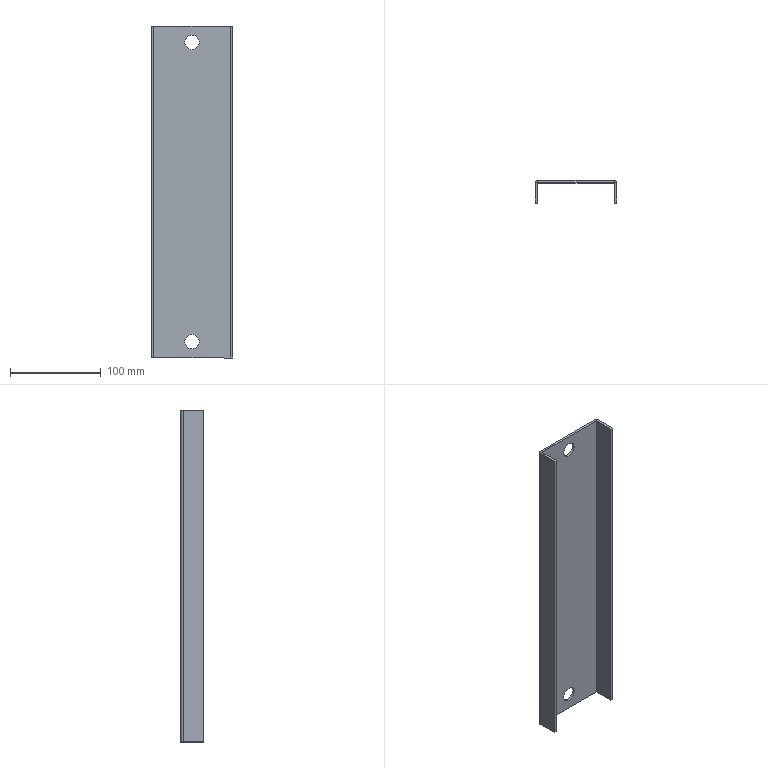Component | SolidWorks | KSHE-016.014-1 | 1 solid | 26 faces | box 90 x 25 x 366 mm | volume 121459 mm3 | plane 18 | cylinder 8 | commonest cylinder face diameters 16 x4 5.2 x2 0.2 x2
STEP:
#1=COLOUR_RGB('',0.7922,0.8196,0.9333);
#2=FILL_AREA_STYLE_COLOUR('',#1);
#3=FILL_AREA_STYLE('',(#2));
#4=SURFACE_STYLE_FILL_AREA(#3);
#5=SURFACE_SIDE_STYLE('',(#4));
#6=SURFACE_STYLE_USAGE(.BOTH.,#5);
#7=PRESENTATION_STYLE_ASSIGNMENT((#6));
#8=CARTESIAN_POINT('',(12.115,67.965,-1.713));
#9=VERTEX_POINT('',#8);
#10=CARTESIAN_POINT('',(12.115,67.965,-2.343));
#11=VERTEX_POINT('',#10);
#12=CARTESIAN_POINT('',(12.115,67.965,-2.028));
#13=DIRECTION('',(0.,1.,-0.));
#14=DIRECTION('',(0.,0.,-1.));
#15=AXIS2_PLACEMENT_3D('',#12,#13,#14);
#16=CIRCLE('',#15,0.315);
#17=EDGE_CURVE('',#9,#11,#16,.T.);
#18=ORIENTED_EDGE('',*,*,#17,.F.);
#19=CARTESIAN_POINT('',(12.115,68.064,-1.713));
#20=VERTEX_POINT('',#19);
#21=CARTESIAN_POINT('',(12.115,67.67,-1.713));
#22=DIRECTION('',(0.,1.,-0.));
#23=VECTOR('',#22,39.37);
#24=LINE('',#21,#23);
#25=EDGE_CURVE('',#9,#20,#24,.T.);
#26=ORIENTED_EDGE('',*,*,#25,.T.);
#27=CARTESIAN_POINT('',(12.115,68.064,-2.343));
#28=VERTEX_POINT('',#27);
#29=CARTESIAN_POINT('',(12.115,68.064,-2.028));
#30=DIRECTION('',(0.,1.,-0.));
#31=DIRECTION('',(0.,0.,-1.));
#32=AXIS2_PLACEMENT_3D('',#29,#30,#31);
#33=CIRCLE('',#32,0.315);
#34=EDGE_CURVE('',#20,#28,#33,.T.);
#35=ORIENTED_EDGE('',*,*,#34,.T.);
#36=CARTESIAN_POINT('',(12.115,67.67,-2.343));
#37=DIRECTION('',(0.,1.,-0.));
#38=VECTOR('',#37,39.37);
#39=LINE('',#36,#38);
#40=EDGE_CURVE('',#11,#28,#39,.T.);
#41=ORIENTED_EDGE('',*,*,#40,.F.);
#42=EDGE_LOOP('',(#18,#26,#35,#41));
#43=FACE_OUTER_BOUND('',#42,.T.);
#44=CARTESIAN_POINT('',(12.115,67.67,-2.028));
#45=DIRECTION('',(0.,1.,-0.));
#46=DIRECTION('',(0.,0.,-1.));
#47=AXIS2_PLACEMENT_3D('',#44,#45,#46);
#48=CYLINDRICAL_SURFACE('',#47,0.315);
#49=ADVANCED_FACE('',(#43),#48,.F.);
#50=CARTESIAN_POINT('',(12.115,67.965,-14.705));
#51=VERTEX_POINT('',#50);
#52=CARTESIAN_POINT('',(12.115,67.965,-15.335));
#53=VERTEX_POINT('',#52);
#54=CARTESIAN_POINT('',(12.115,67.965,-15.02));
#55=DIRECTION('',(0.,1.,-0.));
#56=DIRECTION('',(0.,0.,-1.));
#57=AXIS2_PLACEMENT_3D('',#54,#55,#56);
#58=CIRCLE('',#57,0.315);
#59=EDGE_CURVE('',#51,#53,#58,.T.);
#60=ORIENTED_EDGE('',*,*,#59,.F.);
#61=CARTESIAN_POINT('',(12.115,68.064,-14.705));
#62=VERTEX_POINT('',#61);
#63=CARTESIAN_POINT('',(12.115,67.67,-14.705));
#64=DIRECTION('',(0.,1.,-0.));
#65=VECTOR('',#64,39.37);
#66=LINE('',#63,#65);
#67=EDGE_CURVE('',#51,#62,#66,.T.);
#68=ORIENTED_EDGE('',*,*,#67,.T.);
#69=CARTESIAN_POINT('',(12.115,68.064,-15.335));
#70=VERTEX_POINT('',#69);
#71=CARTESIAN_POINT('',(12.115,68.064,-15.02));
#72=DIRECTION('',(0.,1.,-0.));
#73=DIRECTION('',(0.,0.,-1.));
#74=AXIS2_PLACEMENT_3D('',#71,#72,#73);
#75=CIRCLE('',#74,0.315);
#76=EDGE_CURVE('',#62,#70,#75,.T.);
#77=ORIENTED_EDGE('',*,*,#76,.T.);
#78=CARTESIAN_POINT('',(12.115,67.67,-15.335));
#79=DIRECTION('',(0.,1.,-0.));
#80=VECTOR('',#79,39.37);
#81=LINE('',#78,#80);
#82=EDGE_CURVE('',#53,#70,#81,.T.);
#83=ORIENTED_EDGE('',*,*,#82,.F.);
#84=EDGE_LOOP('',(#60,#68,#77,#83));
#85=FACE_OUTER_BOUND('',#84,.T.);
#86=CARTESIAN_POINT('',(12.115,67.67,-15.02));
#87=DIRECTION('',(0.,1.,-0.));
#88=DIRECTION('',(0.,0.,-1.));
#89=AXIS2_PLACEMENT_3D('',#86,#87,#88);
#90=CYLINDRICAL_SURFACE('',#89,0.315);
#91=ADVANCED_FACE('',(#85),#90,.F.);
#92=CARTESIAN_POINT('',(12.115,67.965,-2.028));
#93=DIRECTION('',(0.,1.,-0.));
#94=DIRECTION('',(0.,0.,-1.));
#95=AXIS2_PLACEMENT_3D('',#92,#93,#94);
#96=CIRCLE('',#95,0.315);
#97=EDGE_CURVE('',#11,#9,#96,.T.);
#98=ORIENTED_EDGE('',*,*,#97,.T.);
#99=ORIENTED_EDGE('',*,*,#17,.T.);
#100=EDGE_LOOP('',(#98,#99));
#101=FACE_BOUND('',#100,.T.);
#102=CARTESIAN_POINT('',(12.115,67.965,-15.02));
#103=DIRECTION('',(0.,1.,-0.));
#104=DIRECTION('',(0.,0.,-1.));
#105=AXIS2_PLACEMENT_3D('',#102,#103,#104);
#106=CIRCLE('',#105,0.315);
#107=EDGE_CURVE('',#53,#51,#106,.T.);
#108=ORIENTED_EDGE('',*,*,#107,.T.);
#109=ORIENTED_EDGE('',*,*,#59,.T.);
#110=EDGE_LOOP('',(#108,#109));
#111=FACE_BOUND('',#110,.T.);
#112=CARTESIAN_POINT('',(13.785,67.965,-1.319));
#113=VERTEX_POINT('',#112);
#114=CARTESIAN_POINT('',(13.785,67.965,-15.728));
#115=VERTEX_POINT('',#114);
#116=CARTESIAN_POINT('',(13.785,67.965,-1.319));
#117=DIRECTION('',(-0.,0.,-1.));
#118=VECTOR('',#117,39.37);
#119=LINE('',#116,#118);
#120=EDGE_CURVE('',#113,#115,#119,.T.);
#121=ORIENTED_EDGE('',*,*,#120,.F.);
#122=CARTESIAN_POINT('',(10.446,67.965,-1.319));
#123=VERTEX_POINT('',#122);
#124=CARTESIAN_POINT('',(10.344,67.965,-1.319));
#125=DIRECTION('',(1.,-0.,-0.));
#126=VECTOR('',#125,39.37);
#127=LINE('',#124,#126);
#128=EDGE_CURVE('',#123,#113,#127,.T.);
#129=ORIENTED_EDGE('',*,*,#128,.F.);
#130=CARTESIAN_POINT('',(10.446,67.965,-15.728));
#131=VERTEX_POINT('',#130);
#132=CARTESIAN_POINT('',(10.446,67.965,-15.728));
#133=DIRECTION('',(0.,-0.,1.));
#134=VECTOR('',#133,39.37);
#135=LINE('',#132,#134);
#136=EDGE_CURVE('',#131,#123,#135,.T.);
#137=ORIENTED_EDGE('',*,*,#136,.F.);
#138=CARTESIAN_POINT('',(10.344,67.965,-15.728));
#139=DIRECTION('',(-1.,0.,0.));
#140=VECTOR('',#139,39.37);
#141=LINE('',#138,#140);
#142=EDGE_CURVE('',#115,#131,#141,.T.);
#143=ORIENTED_EDGE('',*,*,#142,.F.);
#144=EDGE_LOOP('',(#121,#129,#137,#143));
#145=FACE_OUTER_BOUND('',#144,.T.);
#146=CARTESIAN_POINT('',(12.115,67.965,-8.524));
#147=DIRECTION('',(0.,1.,0.));
#148=DIRECTION('',(-0.,0.,-1.));
#149=AXIS2_PLACEMENT_3D('',#146,#147,#148);
#150=PLANE('',#149);
#151=ADVANCED_FACE('',(#101,#111,#145),#150,.F.);
#152=CARTESIAN_POINT('',(12.115,68.064,-2.028));
#153=DIRECTION('',(0.,1.,-0.));
#154=DIRECTION('',(0.,0.,-1.));
#155=AXIS2_PLACEMENT_3D('',#152,#153,#154);
#156=CIRCLE('',#155,0.315);
#157=EDGE_CURVE('',#28,#20,#156,.T.);
#158=ORIENTED_EDGE('',*,*,#157,.F.);
#159=ORIENTED_EDGE('',*,*,#34,.F.);
#160=EDGE_LOOP('',(#158,#159));
#161=FACE_BOUND('',#160,.T.);
#162=CARTESIAN_POINT('',(12.115,68.064,-15.02));
#163=DIRECTION('',(0.,1.,-0.));
#164=DIRECTION('',(0.,0.,-1.));
#165=AXIS2_PLACEMENT_3D('',#162,#163,#164);
#166=CIRCLE('',#165,0.315);
#167=EDGE_CURVE('',#70,#62,#166,.T.);
#168=ORIENTED_EDGE('',*,*,#167,.F.);
#169=ORIENTED_EDGE('',*,*,#76,.F.);
#170=EDGE_LOOP('',(#168,#169));
#171=FACE_BOUND('',#170,.T.);
#172=CARTESIAN_POINT('',(10.446,68.064,-1.319));
#173=VERTEX_POINT('',#172);
#174=CARTESIAN_POINT('',(13.785,68.064,-1.319));
#175=VERTEX_POINT('',#174);
#176=CARTESIAN_POINT('',(10.344,68.064,-1.319));
#177=DIRECTION('',(1.,-0.,-0.));
#178=VECTOR('',#177,39.37);
#179=LINE('',#176,#178);
#180=EDGE_CURVE('',#173,#175,#179,.T.);
#181=ORIENTED_EDGE('',*,*,#180,.T.);
#182=CARTESIAN_POINT('',(13.785,68.064,-15.728));
#183=VERTEX_POINT('',#182);
#184=CARTESIAN_POINT('',(13.785,68.064,-1.319));
#185=DIRECTION('',(-0.,0.,-1.));
#186=VECTOR('',#185,39.37);
#187=LINE('',#184,#186);
#188=EDGE_CURVE('',#175,#183,#187,.T.);
#189=ORIENTED_EDGE('',*,*,#188,.T.);
#190=CARTESIAN_POINT('',(10.446,68.064,-15.728));
#191=VERTEX_POINT('',#190);
#192=CARTESIAN_POINT('',(10.344,68.064,-15.728));
#193=DIRECTION('',(-1.,0.,0.));
#194=VECTOR('',#193,39.37);
#195=LINE('',#192,#194);
#196=EDGE_CURVE('',#183,#191,#195,.T.);
#197=ORIENTED_EDGE('',*,*,#196,.T.);
#198=CARTESIAN_POINT('',(10.446,68.064,-15.728));
#199=DIRECTION('',(0.,-0.,1.));
#200=VECTOR('',#199,39.37);
#201=LINE('',#198,#200);
#202=EDGE_CURVE('',#191,#173,#201,.T.);
#203=ORIENTED_EDGE('',*,*,#202,.T.);
#204=EDGE_LOOP('',(#181,#189,#197,#203));
#205=FACE_OUTER_BOUND('',#204,.T.);
#206=CARTESIAN_POINT('',(12.115,68.064,-8.524));
#207=DIRECTION('',(0.,1.,0.));
#208=DIRECTION('',(-0.,0.,-1.));
#209=AXIS2_PLACEMENT_3D('',#206,#207,#208);
#210=PLANE('',#209);
#211=ADVANCED_FACE('',(#161,#171,#205),#210,.T.);
#212=ORIENTED_EDGE('',*,*,#128,.T.);
#213=CARTESIAN_POINT('',(13.785,67.965,-1.319));
#214=DIRECTION('',(0.,1.,-0.));
#215=VECTOR('',#214,39.37);
#216=LINE('',#213,#215);
#217=EDGE_CURVE('',#113,#175,#216,.T.);
#218=ORIENTED_EDGE('',*,*,#217,.T.);
#219=ORIENTED_EDGE('',*,*,#180,.F.);
#220=CARTESIAN_POINT('',(10.446,67.965,-1.319));
#221=DIRECTION('',(0.,1.,-0.));
#222=VECTOR('',#221,39.37);
#223=LINE('',#220,#222);
#224=EDGE_CURVE('',#123,#173,#223,.T.);
#225=ORIENTED_EDGE('',*,*,#224,.F.);
#226=EDGE_LOOP('',(#212,#218,#219,#225));
#227=FACE_OUTER_BOUND('',#226,.T.);
#228=CARTESIAN_POINT('',(10.344,67.965,-1.319));
#229=DIRECTION('',(0.,0.,1.));
#230=DIRECTION('',(0.,1.,-0.));
#231=AXIS2_PLACEMENT_3D('',#228,#229,#230);
#232=PLANE('',#231);
#233=ADVANCED_FACE('',(#227),#232,.T.);
#234=CARTESIAN_POINT('',(13.785,67.965,-15.728));
#235=DIRECTION('',(0.,1.,-0.));
#236=VECTOR('',#235,39.37);
#237=LINE('',#234,#236);
#238=EDGE_CURVE('',#115,#183,#237,.T.);
#239=ORIENTED_EDGE('',*,*,#238,.F.);
#240=ORIENTED_EDGE('',*,*,#142,.T.);
#241=CARTESIAN_POINT('',(10.446,67.965,-15.728));
#242=DIRECTION('',(0.,1.,-0.));
#243=VECTOR('',#242,39.37);
#244=LINE('',#241,#243);
#245=EDGE_CURVE('',#131,#191,#244,.T.);
#246=ORIENTED_EDGE('',*,*,#245,.T.);
#247=ORIENTED_EDGE('',*,*,#196,.F.);
#248=EDGE_LOOP('',(#239,#240,#246,#247));
#249=FACE_OUTER_BOUND('',#248,.T.);
#250=CARTESIAN_POINT('',(10.344,67.965,-15.728));
#251=DIRECTION('',(-0.,-0.,-1.));
#252=DIRECTION('',(-0.,-1.,0.));
#253=AXIS2_PLACEMENT_3D('',#250,#251,#252);
#254=PLANE('',#253);
#255=ADVANCED_FACE('',(#249),#254,.T.);
#256=CARTESIAN_POINT('',(10.442,67.961,-1.319));
#257=VERTEX_POINT('',#256);
#258=CARTESIAN_POINT('',(10.344,67.961,-1.319));
#259=VERTEX_POINT('',#258);
#260=CARTESIAN_POINT('',(10.344,67.961,-1.319));
#261=DIRECTION('',(-1.,0.,0.));
#262=VECTOR('',#261,39.37);
#263=LINE('',#260,#262);
#264=EDGE_CURVE('',#257,#259,#263,.T.);
#265=ORIENTED_EDGE('',*,*,#264,.F.);
#266=CARTESIAN_POINT('',(10.446,67.961,-1.319));
#267=DIRECTION('',(0.,-0.,1.));
#268=DIRECTION('',(0.,-1.,0.));
#269=AXIS2_PLACEMENT_3D('',#266,#267,#268);
#270=CIRCLE('',#269,0.003937);
#271=EDGE_CURVE('',#123,#257,#270,.T.);
#272=ORIENTED_EDGE('',*,*,#271,.F.);
#273=ORIENTED_EDGE('',*,*,#224,.T.);
#274=CARTESIAN_POINT('',(10.446,67.961,-1.319));
#275=DIRECTION('',(0.,-0.,1.));
#276=DIRECTION('',(0.,-1.,0.));
#277=AXIS2_PLACEMENT_3D('',#274,#275,#276);
#278=CIRCLE('',#277,0.1024);
#279=EDGE_CURVE('',#173,#259,#278,.T.);
#280=ORIENTED_EDGE('',*,*,#279,.T.);
#281=EDGE_LOOP('',(#265,#272,#273,#280));
#282=FACE_OUTER_BOUND('',#281,.T.);
#283=CARTESIAN_POINT('',(10.446,67.961,-1.319));
#284=DIRECTION('',(0.,0.,1.));
#285=DIRECTION('',(0.,1.,-0.));
#286=AXIS2_PLACEMENT_3D('',#283,#284,#285);
#287=PLANE('',#286);
#288=ADVANCED_FACE('',(#282),#287,.T.);
#289=CARTESIAN_POINT('',(10.442,67.961,-15.728));
#290=VERTEX_POINT('',#289);
#291=CARTESIAN_POINT('',(10.446,67.961,-15.728));
#292=DIRECTION('',(-0.,0.,-1.));
#293=DIRECTION('',(0.,-1.,0.));
#294=AXIS2_PLACEMENT_3D('',#291,#292,#293);
#295=CIRCLE('',#294,0.003937);
#296=EDGE_CURVE('',#290,#131,#295,.T.);
#297=ORIENTED_EDGE('',*,*,#296,.F.);
#298=CARTESIAN_POINT('',(10.344,67.961,-15.728));
#299=VERTEX_POINT('',#298);
#300=CARTESIAN_POINT('',(10.442,67.961,-15.728));
#301=DIRECTION('',(-1.,0.,0.));
#302=VECTOR('',#301,39.37);
#303=LINE('',#300,#302);
#304=EDGE_CURVE('',#290,#299,#303,.T.);
#305=ORIENTED_EDGE('',*,*,#304,.T.);
#306=CARTESIAN_POINT('',(10.446,67.961,-15.728));
#307=DIRECTION('',(-0.,0.,-1.));
#308=DIRECTION('',(0.,-1.,0.));
#309=AXIS2_PLACEMENT_3D('',#306,#307,#308);
#310=CIRCLE('',#309,0.1024);
#311=EDGE_CURVE('',#299,#191,#310,.T.);
#312=ORIENTED_EDGE('',*,*,#311,.T.);
#313=ORIENTED_EDGE('',*,*,#245,.F.);
#314=EDGE_LOOP('',(#297,#305,#312,#313));
#315=FACE_OUTER_BOUND('',#314,.T.);
#316=CARTESIAN_POINT('',(10.446,67.961,-15.728));
#317=DIRECTION('',(0.,0.,1.));
#318=DIRECTION('',(0.,1.,-0.));
#319=AXIS2_PLACEMENT_3D('',#316,#317,#318);
#320=PLANE('',#319);
#321=ADVANCED_FACE('',(#315),#320,.F.);
#322=ORIENTED_EDGE('',*,*,#202,.F.);
#323=ORIENTED_EDGE('',*,*,#311,.F.);
#324=CARTESIAN_POINT('',(10.344,67.961,-1.319));
#325=DIRECTION('',(0.,-0.,1.));
#326=VECTOR('',#325,39.37);
#327=LINE('',#324,#326);
#328=EDGE_CURVE('',#299,#259,#327,.T.);
#329=ORIENTED_EDGE('',*,*,#328,.T.);
#330=ORIENTED_EDGE('',*,*,#279,.F.);
#331=EDGE_LOOP('',(#322,#323,#329,#330));
#332=FACE_OUTER_BOUND('',#331,.T.);
#333=CARTESIAN_POINT('',(10.446,67.961,-15.728));
#334=DIRECTION('',(-0.,0.,-1.));
#335=DIRECTION('',(-1.,0.,0.));
#336=AXIS2_PLACEMENT_3D('',#333,#334,#335);
#337=CYLINDRICAL_SURFACE('',#336,0.1024);
#338=ADVANCED_FACE('',(#332),#337,.T.);
#339=ORIENTED_EDGE('',*,*,#136,.T.);
#340=ORIENTED_EDGE('',*,*,#271,.T.);
#341=CARTESIAN_POINT('',(10.442,67.961,-1.319));
#342=DIRECTION('',(-0.,0.,-1.));
#343=VECTOR('',#342,39.37);
#344=LINE('',#341,#343);
#345=EDGE_CURVE('',#257,#290,#344,.T.);
#346=ORIENTED_EDGE('',*,*,#345,.T.);
#347=ORIENTED_EDGE('',*,*,#296,.T.);
#348=EDGE_LOOP('',(#339,#340,#346,#347));
#349=FACE_OUTER_BOUND('',#348,.T.);
#350=CARTESIAN_POINT('',(10.446,67.961,-15.728));
#351=DIRECTION('',(-0.,0.,-1.));
#352=DIRECTION('',(-1.,0.,0.));
#353=AXIS2_PLACEMENT_3D('',#350,#351,#352);
#354=CYLINDRICAL_SURFACE('',#353,0.003937);
#355=ADVANCED_FACE('',(#349),#354,.F.);
#356=ORIENTED_EDGE('',*,*,#304,.F.);
#357=CARTESIAN_POINT('',(10.442,67.079,-15.728));
#358=VERTEX_POINT('',#357);
#359=CARTESIAN_POINT('',(10.442,67.079,-15.728));
#360=DIRECTION('',(-0.,-1.,0.));
#361=VECTOR('',#360,39.37);
#362=LINE('',#359,#361);
#363=EDGE_CURVE('',#290,#358,#362,.T.);
#364=ORIENTED_EDGE('',*,*,#363,.T.);
#365=CARTESIAN_POINT('',(10.344,67.079,-15.728));
#366=VERTEX_POINT('',#365);
#367=CARTESIAN_POINT('',(10.344,67.079,-15.728));
#368=DIRECTION('',(1.,-0.,-0.));
#369=VECTOR('',#368,39.37);
#370=LINE('',#367,#369);
#371=EDGE_CURVE('',#366,#358,#370,.T.);
#372=ORIENTED_EDGE('',*,*,#371,.F.);
#373=CARTESIAN_POINT('',(10.344,68.064,-15.728));
#374=DIRECTION('',(-0.,-1.,0.));
#375=VECTOR('',#374,39.37);
#376=LINE('',#373,#375);
#377=EDGE_CURVE('',#299,#366,#376,.T.);
#378=ORIENTED_EDGE('',*,*,#377,.F.);
#379=EDGE_LOOP('',(#356,#364,#372,#378));
#380=FACE_OUTER_BOUND('',#379,.T.);
#381=CARTESIAN_POINT('',(10.344,67.079,-15.728));
#382=DIRECTION('',(0.,0.,1.));
#383=DIRECTION('',(0.,1.,-0.));
#384=AXIS2_PLACEMENT_3D('',#381,#382,#383);
#385=PLANE('',#384);
#386=ADVANCED_FACE('',(#380),#385,.F.);
#387=ORIENTED_EDGE('',*,*,#264,.T.);
#388=CARTESIAN_POINT('',(10.344,67.079,-1.319));
#389=VERTEX_POINT('',#388);
#390=CARTESIAN_POINT('',(10.344,68.064,-1.319));
#391=DIRECTION('',(0.,1.,-0.));
#392=VECTOR('',#391,39.37);
#393=LINE('',#390,#392);
#394=EDGE_CURVE('',#389,#259,#393,.T.);
#395=ORIENTED_EDGE('',*,*,#394,.F.);
#396=CARTESIAN_POINT('',(10.442,67.079,-1.319));
#397=VERTEX_POINT('',#396);
#398=CARTESIAN_POINT('',(10.344,67.079,-1.319));
#399=DIRECTION('',(1.,-0.,-0.));
#400=VECTOR('',#399,39.37);
#401=LINE('',#398,#400);
#402=EDGE_CURVE('',#389,#397,#401,.T.);
#403=ORIENTED_EDGE('',*,*,#402,.T.);
#404=CARTESIAN_POINT('',(10.442,67.965,-1.319));
#405=DIRECTION('',(0.,1.,-0.));
#406=VECTOR('',#405,39.37);
#407=LINE('',#404,#406);
#408=EDGE_CURVE('',#397,#257,#407,.T.);
#409=ORIENTED_EDGE('',*,*,#408,.T.);
#410=EDGE_LOOP('',(#387,#395,#403,#409));
#411=FACE_OUTER_BOUND('',#410,.T.);
#412=CARTESIAN_POINT('',(10.344,67.965,-1.319));
#413=DIRECTION('',(-0.,-0.,-1.));
#414=DIRECTION('',(-0.,-1.,0.));
#415=AXIS2_PLACEMENT_3D('',#412,#413,#414);
#416=PLANE('',#415);
#417=ADVANCED_FACE('',(#411),#416,.F.);
#418=ORIENTED_EDGE('',*,*,#328,.F.);
#419=ORIENTED_EDGE('',*,*,#377,.T.);
#420=CARTESIAN_POINT('',(10.344,67.079,-8.524));
#421=DIRECTION('',(0.,-0.,1.));
#422=VECTOR('',#421,39.37);
#423=LINE('',#420,#422);
#424=EDGE_CURVE('',#366,#389,#423,.T.);
#425=ORIENTED_EDGE('',*,*,#424,.T.);
#426=ORIENTED_EDGE('',*,*,#394,.T.);
#427=EDGE_LOOP('',(#418,#419,#425,#426));
#428=FACE_OUTER_BOUND('',#427,.T.);
#429=CARTESIAN_POINT('',(10.344,68.064,-8.524));
#430=DIRECTION('',(1.,-0.,-0.));
#431=DIRECTION('',(-0.,-1.,0.));
#432=AXIS2_PLACEMENT_3D('',#429,#430,#431);
#433=PLANE('',#432);
#434=ADVANCED_FACE('',(#428),#433,.F.);
#435=ORIENTED_EDGE('',*,*,#363,.F.);
#436=ORIENTED_EDGE('',*,*,#345,.F.);
#437=ORIENTED_EDGE('',*,*,#408,.F.);
#438=CARTESIAN_POINT('',(10.442,67.079,-1.319));
#439=DIRECTION('',(0.,-0.,1.));
#440=VECTOR('',#439,39.37);
#441=LINE('',#438,#440);
#442=EDGE_CURVE('',#358,#397,#441,.T.);
#443=ORIENTED_EDGE('',*,*,#442,.F.);
#444=EDGE_LOOP('',(#435,#436,#437,#443));
#445=FACE_OUTER_BOUND('',#444,.T.);
#446=CARTESIAN_POINT('',(10.442,68.064,-8.524));
#447=DIRECTION('',(1.,-0.,-0.));
#448=DIRECTION('',(-0.,-1.,0.));
#449=AXIS2_PLACEMENT_3D('',#446,#447,#448);
#450=PLANE('',#449);
#451=ADVANCED_FACE('',(#445),#450,.T.);
#452=ORIENTED_EDGE('',*,*,#442,.T.);
#453=ORIENTED_EDGE('',*,*,#402,.F.);
#454=ORIENTED_EDGE('',*,*,#424,.F.);
#455=ORIENTED_EDGE('',*,*,#371,.T.);
#456=EDGE_LOOP('',(#452,#453,#454,#455));
#457=FACE_OUTER_BOUND('',#456,.T.);
#458=CARTESIAN_POINT('',(10.344,67.079,-1.319));
#459=DIRECTION('',(0.,1.,-0.));
#460=DIRECTION('',(1.,-0.,-0.));
#461=AXIS2_PLACEMENT_3D('',#458,#459,#460);
#462=PLANE('',#461);
#463=ADVANCED_FACE('',(#457),#462,.F.);
#464=CARTESIAN_POINT('',(13.788,67.961,-15.728));
#465=VERTEX_POINT('',#464);
#466=CARTESIAN_POINT('',(13.887,67.961,-15.728));
#467=VERTEX_POINT('',#466);
#468=CARTESIAN_POINT('',(13.887,67.961,-15.728));
#469=DIRECTION('',(1.,-0.,-0.));
#470=VECTOR('',#469,39.37);
#471=LINE('',#468,#470);
#472=EDGE_CURVE('',#465,#467,#471,.T.);
#473=ORIENTED_EDGE('',*,*,#472,.F.);
#474=CARTESIAN_POINT('',(13.785,67.961,-15.728));
#475=DIRECTION('',(-0.,0.,-1.));
#476=DIRECTION('',(0.,1.,0.));
#477=AXIS2_PLACEMENT_3D('',#474,#475,#476);
#478=CIRCLE('',#477,0.003937);
#479=EDGE_CURVE('',#115,#465,#478,.T.);
#480=ORIENTED_EDGE('',*,*,#479,.F.);
#481=ORIENTED_EDGE('',*,*,#238,.T.);
#482=CARTESIAN_POINT('',(13.785,67.961,-15.728));
#483=DIRECTION('',(-0.,0.,-1.));
#484=DIRECTION('',(0.,1.,0.));
#485=AXIS2_PLACEMENT_3D('',#482,#483,#484);
#486=CIRCLE('',#485,0.1024);
#487=EDGE_CURVE('',#183,#467,#486,.T.);
#488=ORIENTED_EDGE('',*,*,#487,.T.);
#489=EDGE_LOOP('',(#473,#480,#481,#488));
#490=FACE_OUTER_BOUND('',#489,.T.);
#491=CARTESIAN_POINT('',(13.785,67.961,-15.728));
#492=DIRECTION('',(-0.,-0.,-1.));
#493=DIRECTION('',(-0.,-1.,0.));
#494=AXIS2_PLACEMENT_3D('',#491,#492,#493);
#495=PLANE('',#494);
#496=ADVANCED_FACE('',(#490),#495,.T.);
#497=CARTESIAN_POINT('',(13.788,67.961,-1.319));
#498=VERTEX_POINT('',#497);
#499=CARTESIAN_POINT('',(13.785,67.961,-1.319));
#500=DIRECTION('',(0.,-0.,1.));
#501=DIRECTION('',(0.,1.,0.));
#502=AXIS2_PLACEMENT_3D('',#499,#500,#501);
#503=CIRCLE('',#502,0.003937);
#504=EDGE_CURVE('',#498,#113,#503,.T.);
#505=ORIENTED_EDGE('',*,*,#504,.F.);
#506=CARTESIAN_POINT('',(13.887,67.961,-1.319));
#507=VERTEX_POINT('',#506);
#508=CARTESIAN_POINT('',(13.788,67.961,-1.319));
#509=DIRECTION('',(1.,-0.,-0.));
#510=VECTOR('',#509,39.37);
#511=LINE('',#508,#510);
#512=EDGE_CURVE('',#498,#507,#511,.T.);
#513=ORIENTED_EDGE('',*,*,#512,.T.);
#514=CARTESIAN_POINT('',(13.785,67.961,-1.319));
#515=DIRECTION('',(0.,-0.,1.));
#516=DIRECTION('',(0.,1.,0.));
#517=AXIS2_PLACEMENT_3D('',#514,#515,#516);
#518=CIRCLE('',#517,0.1024);
#519=EDGE_CURVE('',#507,#175,#518,.T.);
#520=ORIENTED_EDGE('',*,*,#519,.T.);
#521=ORIENTED_EDGE('',*,*,#217,.F.);
#522=EDGE_LOOP('',(#505,#513,#520,#521));
#523=FACE_OUTER_BOUND('',#522,.T.);
#524=CARTESIAN_POINT('',(13.785,67.961,-1.319));
#525=DIRECTION('',(-0.,-0.,-1.));
#526=DIRECTION('',(-0.,-1.,0.));
#527=AXIS2_PLACEMENT_3D('',#524,#525,#526);
#528=PLANE('',#527);
#529=ADVANCED_FACE('',(#523),#528,.F.);
#530=ORIENTED_EDGE('',*,*,#188,.F.);
#531=ORIENTED_EDGE('',*,*,#519,.F.);
#532=CARTESIAN_POINT('',(13.887,67.961,-15.728));
#533=DIRECTION('',(-0.,0.,-1.));
#534=VECTOR('',#533,39.37);
#535=LINE('',#532,#534);
#536=EDGE_CURVE('',#507,#467,#535,.T.);
#537=ORIENTED_EDGE('',*,*,#536,.T.);
#538=ORIENTED_EDGE('',*,*,#487,.F.);
#539=EDGE_LOOP('',(#530,#531,#537,#538));
#540=FACE_OUTER_BOUND('',#539,.T.);
#541=CARTESIAN_POINT('',(13.785,67.961,-1.319));
#542=DIRECTION('',(0.,-0.,1.));
#543=DIRECTION('',(1.,0.,-0.));
#544=AXIS2_PLACEMENT_3D('',#541,#542,#543);
#545=CYLINDRICAL_SURFACE('',#544,0.1024);
#546=ADVANCED_FACE('',(#540),#545,.T.);
#547=ORIENTED_EDGE('',*,*,#120,.T.);
#548=ORIENTED_EDGE('',*,*,#479,.T.);
#549=CARTESIAN_POINT('',(13.788,67.961,-15.728));
#550=DIRECTION('',(0.,-0.,1.));
#551=VECTOR('',#550,39.37);
#552=LINE('',#549,#551);
#553=EDGE_CURVE('',#465,#498,#552,.T.);
#554=ORIENTED_EDGE('',*,*,#553,.T.);
#555=ORIENTED_EDGE('',*,*,#504,.T.);
#556=EDGE_LOOP('',(#547,#548,#554,#555));
#557=FACE_OUTER_BOUND('',#556,.T.);
#558=CARTESIAN_POINT('',(13.785,67.961,-1.319));
#559=DIRECTION('',(0.,-0.,1.));
#560=DIRECTION('',(1.,0.,0.));
#561=AXIS2_PLACEMENT_3D('',#558,#559,#560);
#562=CYLINDRICAL_SURFACE('',#561,0.003937);
#563=ADVANCED_FACE('',(#557),#562,.F.);
#564=ORIENTED_EDGE('',*,*,#512,.F.);
#565=CARTESIAN_POINT('',(13.788,67.079,-1.319));
#566=VERTEX_POINT('',#565);
#567=CARTESIAN_POINT('',(13.788,67.079,-1.319));
#568=DIRECTION('',(-0.,-1.,0.));
#569=VECTOR('',#568,39.37);
#570=LINE('',#567,#569);
#571=EDGE_CURVE('',#498,#566,#570,.T.);
#572=ORIENTED_EDGE('',*,*,#571,.T.);
#573=CARTESIAN_POINT('',(13.887,67.079,-1.319));
#574=VERTEX_POINT('',#573);
#575=CARTESIAN_POINT('',(13.887,67.079,-1.319));
#576=DIRECTION('',(-1.,0.,0.));
#577=VECTOR('',#576,39.37);
#578=LINE('',#575,#577);
#579=EDGE_CURVE('',#574,#566,#578,.T.);
#580=ORIENTED_EDGE('',*,*,#579,.F.);
#581=CARTESIAN_POINT('',(13.887,68.064,-1.319));
#582=DIRECTION('',(-0.,-1.,0.));
#583=VECTOR('',#582,39.37);
#584=LINE('',#581,#583);
#585=EDGE_CURVE('',#507,#574,#584,.T.);
#586=ORIENTED_EDGE('',*,*,#585,.F.);
#587=EDGE_LOOP('',(#564,#572,#580,#586));
#588=FACE_OUTER_BOUND('',#587,.T.);
#589=CARTESIAN_POINT('',(13.887,67.079,-1.319));
#590=DIRECTION('',(-0.,-0.,-1.));
#591=DIRECTION('',(-0.,-1.,0.));
#592=AXIS2_PLACEMENT_3D('',#589,#590,#591);
#593=PLANE('',#592);
#594=ADVANCED_FACE('',(#588),#593,.F.);
#595=ORIENTED_EDGE('',*,*,#472,.T.);
#596=CARTESIAN_POINT('',(13.887,67.079,-15.728));
#597=VERTEX_POINT('',#596);
#598=CARTESIAN_POINT('',(13.887,68.064,-15.728));
#599=DIRECTION('',(0.,1.,-0.));
#600=VECTOR('',#599,39.37);
#601=LINE('',#598,#600);
#602=EDGE_CURVE('',#597,#467,#601,.T.);
#603=ORIENTED_EDGE('',*,*,#602,.F.);
#604=CARTESIAN_POINT('',(13.788,67.079,-15.728));
#605=VERTEX_POINT('',#604);
#606=CARTESIAN_POINT('',(13.887,67.079,-15.728));
#607=DIRECTION('',(-1.,0.,0.));
#608=VECTOR('',#607,39.37);
#609=LINE('',#606,#608);
#610=EDGE_CURVE('',#597,#605,#609,.T.);
#611=ORIENTED_EDGE('',*,*,#610,.T.);
#612=CARTESIAN_POINT('',(13.788,67.965,-15.728));
#613=DIRECTION('',(0.,1.,-0.));
#614=VECTOR('',#613,39.37);
#615=LINE('',#612,#614);
#616=EDGE_CURVE('',#605,#465,#615,.T.);
#617=ORIENTED_EDGE('',*,*,#616,.T.);
#618=EDGE_LOOP('',(#595,#603,#611,#617));
#619=FACE_OUTER_BOUND('',#618,.T.);
#620=CARTESIAN_POINT('',(13.887,67.965,-15.728));
#621=DIRECTION('',(0.,0.,1.));
#622=DIRECTION('',(0.,1.,-0.));
#623=AXIS2_PLACEMENT_3D('',#620,#621,#622);
#624=PLANE('',#623);
#625=ADVANCED_FACE('',(#619),#624,.F.);
#626=ORIENTED_EDGE('',*,*,#536,.F.);
#627=ORIENTED_EDGE('',*,*,#585,.T.);
#628=CARTESIAN_POINT('',(13.887,67.079,-8.524));
#629=DIRECTION('',(-0.,0.,-1.));
#630=VECTOR('',#629,39.37);
#631=LINE('',#628,#630);
#632=EDGE_CURVE('',#574,#597,#631,.T.);
#633=ORIENTED_EDGE('',*,*,#632,.T.);
#634=ORIENTED_EDGE('',*,*,#602,.T.);
#635=EDGE_LOOP('',(#626,#627,#633,#634));
#636=FACE_OUTER_BOUND('',#635,.T.);
#637=CARTESIAN_POINT('',(13.887,68.064,-8.524));
#638=DIRECTION('',(-1.,0.,0.));
#639=DIRECTION('',(0.,1.,-0.));
#640=AXIS2_PLACEMENT_3D('',#637,#638,#639);
#641=PLANE('',#640);
#642=ADVANCED_FACE('',(#636),#641,.F.);
#643=ORIENTED_EDGE('',*,*,#571,.F.);
#644=ORIENTED_EDGE('',*,*,#553,.F.);
#645=ORIENTED_EDGE('',*,*,#616,.F.);
#646=CARTESIAN_POINT('',(13.788,67.079,-15.728));
#647=DIRECTION('',(-0.,0.,-1.));
#648=VECTOR('',#647,39.37);
#649=LINE('',#646,#648);
#650=EDGE_CURVE('',#566,#605,#649,.T.);
#651=ORIENTED_EDGE('',*,*,#650,.F.);
#652=EDGE_LOOP('',(#643,#644,#645,#651));
#653=FACE_OUTER_BOUND('',#652,.T.);
#654=CARTESIAN_POINT('',(13.788,68.064,-8.524));
#655=DIRECTION('',(-1.,0.,0.));
#656=DIRECTION('',(0.,1.,-0.));
#657=AXIS2_PLACEMENT_3D('',#654,#655,#656);
#658=PLANE('',#657);
#659=ADVANCED_FACE('',(#653),#658,.T.);
#660=ORIENTED_EDGE('',*,*,#650,.T.);
#661=ORIENTED_EDGE('',*,*,#610,.F.);
#662=ORIENTED_EDGE('',*,*,#632,.F.);
#663=ORIENTED_EDGE('',*,*,#579,.T.);
#664=EDGE_LOOP('',(#660,#661,#662,#663));
#665=FACE_OUTER_BOUND('',#664,.T.);
#666=CARTESIAN_POINT('',(13.887,67.079,-15.728));
#667=DIRECTION('',(0.,1.,-0.));
#668=DIRECTION('',(1.,-0.,-0.));
#669=AXIS2_PLACEMENT_3D('',#666,#667,#668);
#670=PLANE('',#669);
#671=ADVANCED_FACE('',(#665),#670,.F.);
#672=ORIENTED_EDGE('',*,*,#67,.F.);
#673=ORIENTED_EDGE('',*,*,#107,.F.);
#674=ORIENTED_EDGE('',*,*,#82,.T.);
#675=ORIENTED_EDGE('',*,*,#167,.T.);
#676=EDGE_LOOP('',(#672,#673,#674,#675));
#677=FACE_OUTER_BOUND('',#676,.T.);
#678=CARTESIAN_POINT('',(12.115,67.67,-15.02));
#679=DIRECTION('',(0.,1.,-0.));
#680=DIRECTION('',(0.,0.,-1.));
#681=AXIS2_PLACEMENT_3D('',#678,#679,#680);
#682=CYLINDRICAL_SURFACE('',#681,0.315);
#683=ADVANCED_FACE('',(#677),#682,.F.);
#684=ORIENTED_EDGE('',*,*,#25,.F.);
#685=ORIENTED_EDGE('',*,*,#97,.F.);
#686=ORIENTED_EDGE('',*,*,#40,.T.);
#687=ORIENTED_EDGE('',*,*,#157,.T.);
#688=EDGE_LOOP('',(#684,#685,#686,#687));
#689=FACE_OUTER_BOUND('',#688,.T.);
#690=CARTESIAN_POINT('',(12.115,67.67,-2.028));
#691=DIRECTION('',(0.,1.,-0.));
#692=DIRECTION('',(0.,0.,-1.));
#693=AXIS2_PLACEMENT_3D('',#690,#691,#692);
#694=CYLINDRICAL_SURFACE('',#693,0.315);
#695=ADVANCED_FACE('',(#689),#694,.F.);
#696=CLOSED_SHELL('',(#49,#91,#151,#211,#233,#255,#288,#321,#338,#355,#386,#417,#434,#451,#463,#496,#529,#546,#563,#594,#625,#642,#659,#671,#683,#695));
#697=MANIFOLD_SOLID_BREP('',#696);
#698=STYLED_ITEM('',(#7),#697);
#699=(LENGTH_UNIT()NAMED_UNIT(*)SI_UNIT($,.METRE.));
#700=LENGTH_MEASURE_WITH_UNIT(LENGTH_MEASURE(0.0254),#699);
#701=DIMENSIONAL_EXPONENTS(1.,0.,0.,0.,0.,0.,0.);
#702=(CONVERSION_BASED_UNIT('',#700)LENGTH_UNIT()NAMED_UNIT(#701));
#703=UNCERTAINTY_MEASURE_WITH_UNIT(LENGTH_MEASURE(0.00001),#702,'','');
#704=(NAMED_UNIT(*)PLANE_ANGLE_UNIT()SI_UNIT($,.RADIAN.));
#705=(NAMED_UNIT(*)SI_UNIT($,.STERADIAN.)SOLID_ANGLE_UNIT());
#706=(GEOMETRIC_REPRESENTATION_CONTEXT(3)GLOBAL_UNCERTAINTY_ASSIGNED_CONTEXT((#703))GLOBAL_UNIT_ASSIGNED_CONTEXT((#702,#704,#705))REPRESENTATION_CONTEXT('',''));
#707=MECHANICAL_DESIGN_GEOMETRIC_PRESENTATION_REPRESENTATION('',(#698),#706);
#708=PRESENTATION_LAYER_ASSIGNMENT('','',(#698));
#709=CARTESIAN_POINT('',(0.,0.,0.));
#710=DIRECTION('',(0.,0.,1.));
#711=DIRECTION('',(1.,0.,0.));
#712=AXIS2_PLACEMENT_3D('',#709,#710,#711);
#713=(LENGTH_UNIT()NAMED_UNIT(*)SI_UNIT($,.METRE.));
#714=LENGTH_MEASURE_WITH_UNIT(LENGTH_MEASURE(0.0254),#713);
#715=DIMENSIONAL_EXPONENTS(1.,0.,0.,0.,0.,0.,0.);
#716=(CONVERSION_BASED_UNIT('',#714)LENGTH_UNIT()NAMED_UNIT(#715));
#717=UNCERTAINTY_MEASURE_WITH_UNIT(LENGTH_MEASURE(0.00001),#716,'','');
#718=(NAMED_UNIT(*)PLANE_ANGLE_UNIT()SI_UNIT($,.RADIAN.));
#719=(NAMED_UNIT(*)SI_UNIT($,.STERADIAN.)SOLID_ANGLE_UNIT());
#720=(GEOMETRIC_REPRESENTATION_CONTEXT(3)GLOBAL_UNCERTAINTY_ASSIGNED_CONTEXT((#717))GLOBAL_UNIT_ASSIGNED_CONTEXT((#716,#718,#719))REPRESENTATION_CONTEXT('',''));
#721=ADVANCED_BREP_SHAPE_REPRESENTATION('',(#697,#712),#720);